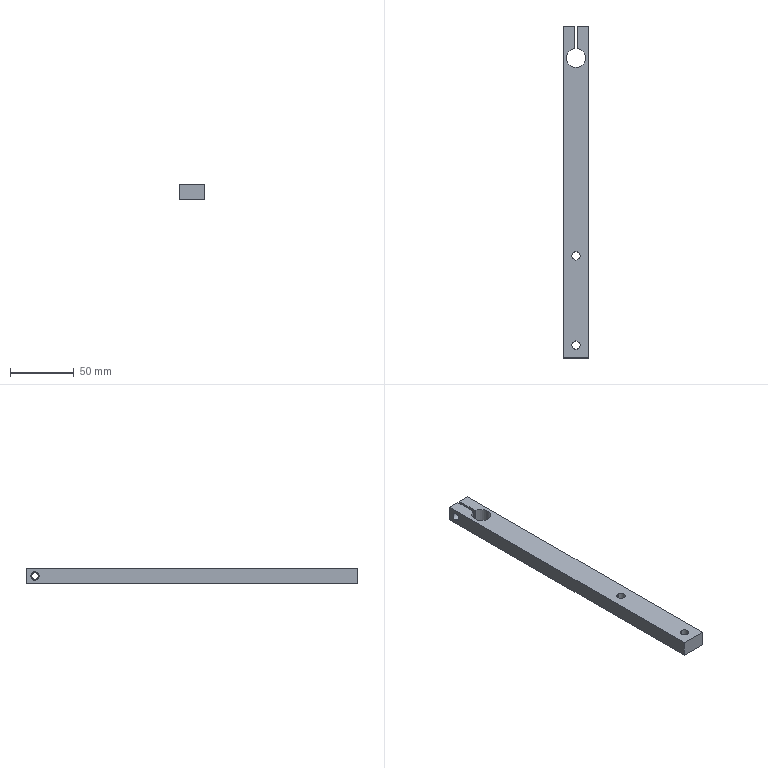Component | SolidWorks | KSD171005A-01-01-23-1 | 1 solid | 24 faces | box 20 x 260 x 12 mm | volume 57833 mm3 | cylinder 13 | plane 11 | commonest cylinder face diameters 11 x4 6.6 x4 6.5 x2 5 x2 15 x1
build123d program:
from build123d import *

# Parameters (mm, degrees)
SKETCH1_W                                       = 260
SKETCH1_H                                       = 20
BOSS_EXTRUDE1_DEPTH                             = 12
SKETCH2_R                                       = 7.5
CUT_EXTRUDE1_DEPTH                              = 131.935
SKETCH3_W                                       = 20
SKETCH3_H                                       = 2
CUT_EXTRUDE2_DEPTH                              = 131.935
M6_TAPPED_HOLE1_D                               = 5
F_6_5_6_5_DIAMETER_HOLE1_D                      = 6.5
F_6_5_6_5_DIAMETER_HOLE1_DEPTH                  = 10
F_6_5_6_5_DIAMETER_HOLE1_TIP                    = 1.953
M6_HEX_SOCKET_HEAD_CAP_SCREW_CBORE2_D           = 6.6
M6_HEX_SOCKET_HEAD_CAP_SCREW_CBORE2_CBORE_D     = 11
M6_HEX_SOCKET_HEAD_CAP_SCREW_CBORE2_CBORE_DEPTH = 6


with BuildPart() as part:
    # Sketch1 → Boss-Extrude1 (new body)
    with BuildSketch(Plane.XY):
        Rectangle(SKETCH1_W, SKETCH1_H)
    extrude(amount=BOSS_EXTRUDE1_DEPTH)

    # Sketch2 → Cut-Extrude1 (cut, through all)
    with BuildSketch(Plane.XY.offset(12)):
        with Locations((105, 0)):
            Circle(SKETCH2_R)
    extrude(amount=-CUT_EXTRUDE1_DEPTH, mode=Mode.SUBTRACT)

    # Sketch3 → Cut-Extrude2 (cut, through all)
    with BuildSketch(Plane.XY.offset(12)):
        with Locations((120, 0)):
            Rectangle(SKETCH3_W, SKETCH3_H)
    extrude(amount=-CUT_EXTRUDE2_DEPTH, mode=Mode.SUBTRACT)

    # M6 Tapped Hole1 (through all)
    with Locations(Plane(origin=(0, 10, 0), x_dir=(1, 0, 0), z_dir=(0, 1, 0))):
        with Locations((123, -6)):
            Hole(M6_TAPPED_HOLE1_D / 2)

    # 6.5 _6.5_ Diameter Hole1
    with Locations(Plane(origin=(0, 10, 0), x_dir=(1, 0, 0), z_dir=(0, 1, 0))):
        with Locations((123, -6)):
            Hole(F_6_5_6_5_DIAMETER_HOLE1_D / 2, depth=F_6_5_6_5_DIAMETER_HOLE1_DEPTH)
            with Locations((0, 0, -(F_6_5_6_5_DIAMETER_HOLE1_DEPTH + F_6_5_6_5_DIAMETER_HOLE1_TIP / 2))):  # 118° drill point
                Cone(0, F_6_5_6_5_DIAMETER_HOLE1_D / 2, F_6_5_6_5_DIAMETER_HOLE1_TIP, mode=Mode.SUBTRACT)

    # M6 Hex Socket Head Cap Screw CBORE2 (through all)
    with Locations(Plane(origin=(0, 0, 0), x_dir=(-1, 0, 0), z_dir=(0, 0, -1))):
        with Locations((120, 0), (50, 0)):
            CounterBoreHole(M6_HEX_SOCKET_HEAD_CAP_SCREW_CBORE2_D / 2, M6_HEX_SOCKET_HEAD_CAP_SCREW_CBORE2_CBORE_D / 2, M6_HEX_SOCKET_HEAD_CAP_SCREW_CBORE2_CBORE_DEPTH)


solid = part.part

# Placed as in the assembly
solid = solid.moved(Location((-7.111, -89.27, 616), (0, 0, 90)))
STEP:
#1=CARTESIAN_POINT('',(-0.28,-8.022,24.488));
#2=VERTEX_POINT('',#1);
#3=CARTESIAN_POINT('',(-0.28,-8.456,24.488));
#4=VERTEX_POINT('',#3);
#5=CARTESIAN_POINT('',(-0.28,-8.239,24.488));
#6=DIRECTION('',(0.,0.,-1.));
#7=DIRECTION('',(-0.,-1.,0.));
#8=AXIS2_PLACEMENT_3D('',#5,#6,#7);
#9=CIRCLE('',#8,0.2165);
#10=EDGE_CURVE('',#2,#4,#9,.T.);
#11=ORIENTED_EDGE('',*,*,#10,.F.);
#12=CARTESIAN_POINT('',(-0.28,-8.022,24.252));
#13=VERTEX_POINT('',#12);
#14=CARTESIAN_POINT('',(-0.28,-8.022,24.252));
#15=DIRECTION('',(0.,0.,-1.));
#16=VECTOR('',#15,39.37);
#17=LINE('',#14,#16);
#18=EDGE_CURVE('',#2,#13,#17,.T.);
#19=ORIENTED_EDGE('',*,*,#18,.T.);
#20=CARTESIAN_POINT('',(-0.28,-8.456,24.252));
#21=VERTEX_POINT('',#20);
#22=CARTESIAN_POINT('',(-0.28,-8.239,24.252));
#23=DIRECTION('',(0.,0.,-1.));
#24=DIRECTION('',(-0.,-1.,0.));
#25=AXIS2_PLACEMENT_3D('',#22,#23,#24);
#26=CIRCLE('',#25,0.2165);
#27=EDGE_CURVE('',#13,#21,#26,.T.);
#28=ORIENTED_EDGE('',*,*,#27,.T.);
#29=CARTESIAN_POINT('',(-0.28,-8.456,24.252));
#30=DIRECTION('',(0.,0.,-1.));
#31=VECTOR('',#30,39.37);
#32=LINE('',#29,#31);
#33=EDGE_CURVE('',#4,#21,#32,.T.);
#34=ORIENTED_EDGE('',*,*,#33,.F.);
#35=EDGE_LOOP('',(#11,#19,#28,#34));
#36=FACE_OUTER_BOUND('',#35,.T.);
#37=CARTESIAN_POINT('',(-0.28,-8.239,24.252));
#38=DIRECTION('',(0.,0.,-1.));
#39=DIRECTION('',(-0.,-1.,0.));
#40=AXIS2_PLACEMENT_3D('',#37,#38,#39);
#41=CYLINDRICAL_SURFACE('',#40,0.2165);
#42=ADVANCED_FACE('',(#36),#41,.F.);
#43=CARTESIAN_POINT('',(-0.28,-8.109,24.724));
#44=VERTEX_POINT('',#43);
#45=CARTESIAN_POINT('',(-0.28,-8.369,24.724));
#46=VERTEX_POINT('',#45);
#47=CARTESIAN_POINT('',(-0.28,-8.239,24.724));
#48=DIRECTION('',(0.,0.,-1.));
#49=DIRECTION('',(-0.,-1.,0.));
#50=AXIS2_PLACEMENT_3D('',#47,#48,#49);
#51=CIRCLE('',#50,0.1299);
#52=EDGE_CURVE('',#44,#46,#51,.T.);
#53=ORIENTED_EDGE('',*,*,#52,.F.);
#54=CARTESIAN_POINT('',(-0.28,-8.109,24.488));
#55=VERTEX_POINT('',#54);
#56=CARTESIAN_POINT('',(-0.28,-8.109,24.252));
#57=DIRECTION('',(0.,0.,-1.));
#58=VECTOR('',#57,39.37);
#59=LINE('',#56,#58);
#60=EDGE_CURVE('',#44,#55,#59,.T.);
#61=ORIENTED_EDGE('',*,*,#60,.T.);
#62=CARTESIAN_POINT('',(-0.28,-8.369,24.488));
#63=VERTEX_POINT('',#62);
#64=CARTESIAN_POINT('',(-0.28,-8.239,24.488));
#65=DIRECTION('',(0.,0.,-1.));
#66=DIRECTION('',(-0.,-1.,0.));
#67=AXIS2_PLACEMENT_3D('',#64,#65,#66);
#68=CIRCLE('',#67,0.1299);
#69=EDGE_CURVE('',#55,#63,#68,.T.);
#70=ORIENTED_EDGE('',*,*,#69,.T.);
#71=CARTESIAN_POINT('',(-0.28,-8.369,24.252));
#72=DIRECTION('',(0.,0.,-1.));
#73=VECTOR('',#72,39.37);
#74=LINE('',#71,#73);
#75=EDGE_CURVE('',#46,#63,#74,.T.);
#76=ORIENTED_EDGE('',*,*,#75,.F.);
#77=EDGE_LOOP('',(#53,#61,#70,#76));
#78=FACE_OUTER_BOUND('',#77,.T.);
#79=CARTESIAN_POINT('',(-0.28,-8.239,24.252));
#80=DIRECTION('',(0.,0.,-1.));
#81=DIRECTION('',(-0.,-1.,0.));
#82=AXIS2_PLACEMENT_3D('',#79,#80,#81);
#83=CYLINDRICAL_SURFACE('',#82,0.1299);
#84=ADVANCED_FACE('',(#78),#83,.F.);
#85=CARTESIAN_POINT('',(-0.28,-5.267,24.488));
#86=VERTEX_POINT('',#85);
#87=CARTESIAN_POINT('',(-0.28,-5.7,24.488));
#88=VERTEX_POINT('',#87);
#89=CARTESIAN_POINT('',(-0.28,-5.483,24.488));
#90=DIRECTION('',(0.,0.,-1.));
#91=DIRECTION('',(-0.,-1.,0.));
#92=AXIS2_PLACEMENT_3D('',#89,#90,#91);
#93=CIRCLE('',#92,0.2165);
#94=EDGE_CURVE('',#86,#88,#93,.T.);
#95=ORIENTED_EDGE('',*,*,#94,.F.);
#96=CARTESIAN_POINT('',(-0.28,-5.267,24.252));
#97=VERTEX_POINT('',#96);
#98=CARTESIAN_POINT('',(-0.28,-5.267,24.252));
#99=DIRECTION('',(0.,0.,-1.));
#100=VECTOR('',#99,39.37);
#101=LINE('',#98,#100);
#102=EDGE_CURVE('',#86,#97,#101,.T.);
#103=ORIENTED_EDGE('',*,*,#102,.T.);
#104=CARTESIAN_POINT('',(-0.28,-5.7,24.252));
#105=VERTEX_POINT('',#104);
#106=CARTESIAN_POINT('',(-0.28,-5.483,24.252));
#107=DIRECTION('',(0.,0.,-1.));
#108=DIRECTION('',(-0.,-1.,0.));
#109=AXIS2_PLACEMENT_3D('',#106,#107,#108);
#110=CIRCLE('',#109,0.2165);
#111=EDGE_CURVE('',#97,#105,#110,.T.);
#112=ORIENTED_EDGE('',*,*,#111,.T.);
#113=CARTESIAN_POINT('',(-0.28,-5.7,24.252));
#114=DIRECTION('',(0.,0.,-1.));
#115=VECTOR('',#114,39.37);
#116=LINE('',#113,#115);
#117=EDGE_CURVE('',#88,#105,#116,.T.);
#118=ORIENTED_EDGE('',*,*,#117,.F.);
#119=EDGE_LOOP('',(#95,#103,#112,#118));
#120=FACE_OUTER_BOUND('',#119,.T.);
#121=CARTESIAN_POINT('',(-0.28,-5.483,24.252));
#122=DIRECTION('',(0.,0.,-1.));
#123=DIRECTION('',(-0.,-1.,0.));
#124=AXIS2_PLACEMENT_3D('',#121,#122,#123);
#125=CYLINDRICAL_SURFACE('',#124,0.2165);
#126=ADVANCED_FACE('',(#120),#125,.F.);
#127=CARTESIAN_POINT('',(-0.28,-5.353,24.724));
#128=VERTEX_POINT('',#127);
#129=CARTESIAN_POINT('',(-0.28,-5.613,24.724));
#130=VERTEX_POINT('',#129);
#131=CARTESIAN_POINT('',(-0.28,-5.483,24.724));
#132=DIRECTION('',(0.,0.,-1.));
#133=DIRECTION('',(-0.,-1.,0.));
#134=AXIS2_PLACEMENT_3D('',#131,#132,#133);
#135=CIRCLE('',#134,0.1299);
#136=EDGE_CURVE('',#128,#130,#135,.T.);
#137=ORIENTED_EDGE('',*,*,#136,.F.);
#138=CARTESIAN_POINT('',(-0.28,-5.353,24.488));
#139=VERTEX_POINT('',#138);
#140=CARTESIAN_POINT('',(-0.28,-5.353,24.252));
#141=DIRECTION('',(0.,0.,-1.));
#142=VECTOR('',#141,39.37);
#143=LINE('',#140,#142);
#144=EDGE_CURVE('',#128,#139,#143,.T.);
#145=ORIENTED_EDGE('',*,*,#144,.T.);
#146=CARTESIAN_POINT('',(-0.28,-5.613,24.488));
#147=VERTEX_POINT('',#146);
#148=CARTESIAN_POINT('',(-0.28,-5.483,24.488));
#149=DIRECTION('',(0.,0.,-1.));
#150=DIRECTION('',(-0.,-1.,0.));
#151=AXIS2_PLACEMENT_3D('',#148,#149,#150);
#152=CIRCLE('',#151,0.1299);
#153=EDGE_CURVE('',#139,#147,#152,.T.);
#154=ORIENTED_EDGE('',*,*,#153,.T.);
#155=CARTESIAN_POINT('',(-0.28,-5.613,24.252));
#156=DIRECTION('',(0.,0.,-1.));
#157=VECTOR('',#156,39.37);
#158=LINE('',#155,#157);
#159=EDGE_CURVE('',#130,#147,#158,.T.);
#160=ORIENTED_EDGE('',*,*,#159,.F.);
#161=EDGE_LOOP('',(#137,#145,#154,#160));
#162=FACE_OUTER_BOUND('',#161,.T.);
#163=CARTESIAN_POINT('',(-0.28,-5.483,24.252));
#164=DIRECTION('',(0.,0.,-1.));
#165=DIRECTION('',(-0.,-1.,0.));
#166=AXIS2_PLACEMENT_3D('',#163,#164,#165);
#167=CYLINDRICAL_SURFACE('',#166,0.1299);
#168=ADVANCED_FACE('',(#162),#167,.F.);
#169=CARTESIAN_POINT('',(-0.3193,1.328,24.36));
#170=VERTEX_POINT('',#169);
#171=CARTESIAN_POINT('',(-0.3193,1.328,24.616));
#172=VERTEX_POINT('',#171);
#173=CARTESIAN_POINT('',(-0.3193,1.328,24.488));
#174=DIRECTION('',(-1.,0.,0.));
#175=DIRECTION('',(0.,-1.,0.));
#176=AXIS2_PLACEMENT_3D('',#173,#174,#175);
#177=CIRCLE('',#176,0.128);
#178=EDGE_CURVE('',#170,#172,#177,.T.);
#179=ORIENTED_EDGE('',*,*,#178,.F.);
#180=CARTESIAN_POINT('',(-0.6737,1.328,24.36));
#181=VERTEX_POINT('',#180);
#182=CARTESIAN_POINT('',(-0.6737,1.328,24.36));
#183=DIRECTION('',(-1.,0.,0.));
#184=VECTOR('',#183,39.37);
#185=LINE('',#182,#184);
#186=EDGE_CURVE('',#170,#181,#185,.T.);
#187=ORIENTED_EDGE('',*,*,#186,.T.);
#188=CARTESIAN_POINT('',(-0.6737,1.328,24.616));
#189=VERTEX_POINT('',#188);
#190=CARTESIAN_POINT('',(-0.6737,1.328,24.488));
#191=DIRECTION('',(-1.,0.,0.));
#192=DIRECTION('',(0.,0.,1.));
#193=AXIS2_PLACEMENT_3D('',#190,#191,#192);
#194=CIRCLE('',#193,0.128);
#195=EDGE_CURVE('',#181,#189,#194,.T.);
#196=ORIENTED_EDGE('',*,*,#195,.T.);
#197=CARTESIAN_POINT('',(-0.6737,1.328,24.616));
#198=DIRECTION('',(-1.,0.,0.));
#199=VECTOR('',#198,39.37);
#200=LINE('',#197,#199);
#201=EDGE_CURVE('',#172,#189,#200,.T.);
#202=ORIENTED_EDGE('',*,*,#201,.F.);
#203=EDGE_LOOP('',(#179,#187,#196,#202));
#204=FACE_OUTER_BOUND('',#203,.T.);
#205=CARTESIAN_POINT('',(-0.6737,1.328,24.488));
#206=DIRECTION('',(-1.,0.,0.));
#207=DIRECTION('',(0.,0.,1.));
#208=AXIS2_PLACEMENT_3D('',#205,#206,#207);
#209=CYLINDRICAL_SURFACE('',#208,0.128);
#210=ADVANCED_FACE('',(#204),#209,.F.);
#211=CARTESIAN_POINT('',(0.1137,1.328,24.39));
#212=VERTEX_POINT('',#211);
#213=CARTESIAN_POINT('',(0.1137,1.328,24.587));
#214=VERTEX_POINT('',#213);
#215=CARTESIAN_POINT('',(0.1137,1.328,24.488));
#216=DIRECTION('',(-1.,0.,0.));
#217=DIRECTION('',(0.,0.,1.));
#218=AXIS2_PLACEMENT_3D('',#215,#216,#217);
#219=CIRCLE('',#218,0.09843);
#220=EDGE_CURVE('',#212,#214,#219,.T.);
#221=ORIENTED_EDGE('',*,*,#220,.F.);
#222=CARTESIAN_POINT('',(-0.2406,1.328,24.39));
#223=VERTEX_POINT('',#222);
#224=CARTESIAN_POINT('',(-0.6737,1.328,24.39));
#225=DIRECTION('',(-1.,0.,0.));
#226=VECTOR('',#225,39.37);
#227=LINE('',#224,#226);
#228=EDGE_CURVE('',#212,#223,#227,.T.);
#229=ORIENTED_EDGE('',*,*,#228,.T.);
#230=CARTESIAN_POINT('',(-0.2406,1.328,24.587));
#231=VERTEX_POINT('',#230);
#232=CARTESIAN_POINT('',(-0.2406,1.328,24.488));
#233=DIRECTION('',(1.,-0.,0.));
#234=DIRECTION('',(0.,1.,0.));
#235=AXIS2_PLACEMENT_3D('',#232,#233,#234);
#236=CIRCLE('',#235,0.09843);
#237=EDGE_CURVE('',#231,#223,#236,.T.);
#238=ORIENTED_EDGE('',*,*,#237,.F.);
#239=CARTESIAN_POINT('',(-0.6737,1.328,24.587));
#240=DIRECTION('',(-1.,0.,0.));
#241=VECTOR('',#240,39.37);
#242=LINE('',#239,#241);
#243=EDGE_CURVE('',#214,#231,#242,.T.);
#244=ORIENTED_EDGE('',*,*,#243,.F.);
#245=EDGE_LOOP('',(#221,#229,#238,#244));
#246=FACE_OUTER_BOUND('',#245,.T.);
#247=CARTESIAN_POINT('',(-0.6737,1.328,24.488));
#248=DIRECTION('',(-1.,0.,0.));
#249=DIRECTION('',(0.,0.,1.));
#250=AXIS2_PLACEMENT_3D('',#247,#248,#249);
#251=CYLINDRICAL_SURFACE('',#250,0.09843);
#252=ADVANCED_FACE('',(#246),#251,.F.);
#253=CARTESIAN_POINT('',(-0.3193,1.604,24.724));
#254=VERTEX_POINT('',#253);
#255=CARTESIAN_POINT('',(-0.6737,1.604,24.724));
#256=VERTEX_POINT('',#255);
#257=CARTESIAN_POINT('',(-0.6737,1.604,24.724));
#258=DIRECTION('',(-1.,0.,0.));
#259=VECTOR('',#258,39.37);
#260=LINE('',#257,#259);
#261=EDGE_CURVE('',#254,#256,#260,.T.);
#262=ORIENTED_EDGE('',*,*,#261,.F.);
#263=CARTESIAN_POINT('',(-0.3193,1.604,24.252));
#264=VERTEX_POINT('',#263);
#265=CARTESIAN_POINT('',(-0.3193,1.604,24.252));
#266=DIRECTION('',(0.,0.,1.));
#267=VECTOR('',#266,39.37);
#268=LINE('',#265,#267);
#269=EDGE_CURVE('',#264,#254,#268,.T.);
#270=ORIENTED_EDGE('',*,*,#269,.F.);
#271=CARTESIAN_POINT('',(-0.6737,1.604,24.252));
#272=VERTEX_POINT('',#271);
#273=CARTESIAN_POINT('',(-0.6737,1.604,24.252));
#274=DIRECTION('',(-1.,0.,0.));
#275=VECTOR('',#274,39.37);
#276=LINE('',#273,#275);
#277=EDGE_CURVE('',#264,#272,#276,.T.);
#278=ORIENTED_EDGE('',*,*,#277,.T.);
#279=CARTESIAN_POINT('',(-0.6737,1.604,24.724));
#280=DIRECTION('',(0.,0.,-1.));
#281=VECTOR('',#280,39.37);
#282=LINE('',#279,#281);
#283=EDGE_CURVE('',#256,#272,#282,.T.);
#284=ORIENTED_EDGE('',*,*,#283,.F.);
#285=EDGE_LOOP('',(#262,#270,#278,#284));
#286=FACE_OUTER_BOUND('',#285,.T.);
#287=CARTESIAN_POINT('',(-0.6737,1.604,24.724));
#288=DIRECTION('',(-0.,-1.,0.));
#289=DIRECTION('',(0.,0.,1.));
#290=AXIS2_PLACEMENT_3D('',#287,#288,#289);
#291=PLANE('',#290);
#292=ADVANCED_FACE('',(#286),#291,.F.);
#293=CARTESIAN_POINT('',(0.1137,1.604,24.252));
#294=VERTEX_POINT('',#293);
#295=CARTESIAN_POINT('',(-0.2406,1.604,24.252));
#296=VERTEX_POINT('',#295);
#297=CARTESIAN_POINT('',(-0.6737,1.604,24.252));
#298=DIRECTION('',(-1.,0.,0.));
#299=VECTOR('',#298,39.37);
#300=LINE('',#297,#299);
#301=EDGE_CURVE('',#294,#296,#300,.T.);
#302=ORIENTED_EDGE('',*,*,#301,.T.);
#303=CARTESIAN_POINT('',(-0.2406,1.604,24.724));
#304=VERTEX_POINT('',#303);
#305=CARTESIAN_POINT('',(-0.2406,1.604,24.252));
#306=DIRECTION('',(0.,0.,1.));
#307=VECTOR('',#306,39.37);
#308=LINE('',#305,#307);
#309=EDGE_CURVE('',#296,#304,#308,.T.);
#310=ORIENTED_EDGE('',*,*,#309,.T.);
#311=CARTESIAN_POINT('',(0.1137,1.604,24.724));
#312=VERTEX_POINT('',#311);
#313=CARTESIAN_POINT('',(-0.6737,1.604,24.724));
#314=DIRECTION('',(-1.,0.,0.));
#315=VECTOR('',#314,39.37);
#316=LINE('',#313,#315);
#317=EDGE_CURVE('',#312,#304,#316,.T.);
#318=ORIENTED_EDGE('',*,*,#317,.F.);
#319=CARTESIAN_POINT('',(0.1137,1.604,24.724));
#320=DIRECTION('',(0.,0.,-1.));
#321=VECTOR('',#320,39.37);
#322=LINE('',#319,#321);
#323=EDGE_CURVE('',#312,#294,#322,.T.);
#324=ORIENTED_EDGE('',*,*,#323,.T.);
#325=EDGE_LOOP('',(#302,#310,#318,#324));
#326=FACE_OUTER_BOUND('',#325,.T.);
#327=CARTESIAN_POINT('',(-0.6737,1.604,24.724));
#328=DIRECTION('',(-0.,-1.,0.));
#329=DIRECTION('',(0.,0.,1.));
#330=AXIS2_PLACEMENT_3D('',#327,#328,#329);
#331=PLANE('',#330);
#332=ADVANCED_FACE('',(#326),#331,.F.);
#333=CARTESIAN_POINT('',(-0.6737,1.328,24.488));
#334=DIRECTION('',(-1.,0.,0.));
#335=DIRECTION('',(0.,0.,1.));
#336=AXIS2_PLACEMENT_3D('',#333,#334,#335);
#337=CIRCLE('',#336,0.128);
#338=EDGE_CURVE('',#189,#181,#337,.T.);
#339=ORIENTED_EDGE('',*,*,#338,.F.);
#340=ORIENTED_EDGE('',*,*,#195,.F.);
#341=EDGE_LOOP('',(#339,#340));
#342=FACE_BOUND('',#341,.T.);
#343=CARTESIAN_POINT('',(-0.6737,-8.633,24.252));
#344=VERTEX_POINT('',#343);
#345=CARTESIAN_POINT('',(-0.6737,-8.633,24.252));
#346=DIRECTION('',(-0.,-1.,0.));
#347=VECTOR('',#346,39.37);
#348=LINE('',#345,#347);
#349=EDGE_CURVE('',#272,#344,#348,.T.);
#350=ORIENTED_EDGE('',*,*,#349,.T.);
#351=CARTESIAN_POINT('',(-0.6737,-8.633,24.724));
#352=VERTEX_POINT('',#351);
#353=CARTESIAN_POINT('',(-0.6737,-8.633,24.724));
#354=DIRECTION('',(0.,0.,-1.));
#355=VECTOR('',#354,39.37);
#356=LINE('',#353,#355);
#357=EDGE_CURVE('',#352,#344,#356,.T.);
#358=ORIENTED_EDGE('',*,*,#357,.F.);
#359=CARTESIAN_POINT('',(-0.6737,-8.633,24.724));
#360=DIRECTION('',(-0.,-1.,0.));
#361=VECTOR('',#360,39.37);
#362=LINE('',#359,#361);
#363=EDGE_CURVE('',#256,#352,#362,.T.);
#364=ORIENTED_EDGE('',*,*,#363,.F.);
#365=ORIENTED_EDGE('',*,*,#283,.T.);
#366=EDGE_LOOP('',(#350,#358,#364,#365));
#367=FACE_OUTER_BOUND('',#366,.T.);
#368=CARTESIAN_POINT('',(-0.6737,-8.633,24.724));
#369=DIRECTION('',(1.,-0.,0.));
#370=DIRECTION('',(0.,0.,-1.));
#371=AXIS2_PLACEMENT_3D('',#368,#369,#370);
#372=PLANE('',#371);
#373=ADVANCED_FACE('',(#342,#367),#372,.F.);
#374=CARTESIAN_POINT('',(0.1137,-8.633,24.252));
#375=VERTEX_POINT('',#374);
#376=CARTESIAN_POINT('',(-0.6737,-8.633,24.252));
#377=DIRECTION('',(1.,-0.,0.));
#378=VECTOR('',#377,39.37);
#379=LINE('',#376,#378);
#380=EDGE_CURVE('',#344,#375,#379,.T.);
#381=ORIENTED_EDGE('',*,*,#380,.T.);
#382=CARTESIAN_POINT('',(0.1137,-8.633,24.724));
#383=VERTEX_POINT('',#382);
#384=CARTESIAN_POINT('',(0.1137,-8.633,24.724));
#385=DIRECTION('',(0.,0.,-1.));
#386=VECTOR('',#385,39.37);
#387=LINE('',#384,#386);
#388=EDGE_CURVE('',#383,#375,#387,.T.);
#389=ORIENTED_EDGE('',*,*,#388,.F.);
#390=CARTESIAN_POINT('',(-0.6737,-8.633,24.724));
#391=DIRECTION('',(1.,-0.,0.));
#392=VECTOR('',#391,39.37);
#393=LINE('',#390,#392);
#394=EDGE_CURVE('',#352,#383,#393,.T.);
#395=ORIENTED_EDGE('',*,*,#394,.F.);
#396=ORIENTED_EDGE('',*,*,#357,.T.);
#397=EDGE_LOOP('',(#381,#389,#395,#396));
#398=FACE_OUTER_BOUND('',#397,.T.);
#399=CARTESIAN_POINT('',(-0.6737,-8.633,24.724));
#400=DIRECTION('',(0.,1.,0.));
#401=DIRECTION('',(0.,0.,-1.));
#402=AXIS2_PLACEMENT_3D('',#399,#400,#401);
#403=PLANE('',#402);
#404=ADVANCED_FACE('',(#398),#403,.F.);
#405=CARTESIAN_POINT('',(0.1137,1.328,24.488));
#406=DIRECTION('',(-1.,0.,0.));
#407=DIRECTION('',(0.,0.,1.));
#408=AXIS2_PLACEMENT_3D('',#405,#406,#407);
#409=CIRCLE('',#408,0.09843);
#410=EDGE_CURVE('',#214,#212,#409,.T.);
#411=ORIENTED_EDGE('',*,*,#410,.T.);
#412=ORIENTED_EDGE('',*,*,#220,.T.);
#413=EDGE_LOOP('',(#411,#412));
#414=FACE_BOUND('',#413,.T.);
#415=CARTESIAN_POINT('',(0.1137,-8.633,24.252));
#416=DIRECTION('',(0.,1.,0.));
#417=VECTOR('',#416,39.37);
#418=LINE('',#415,#417);
#419=EDGE_CURVE('',#375,#294,#418,.T.);
#420=ORIENTED_EDGE('',*,*,#419,.T.);
#421=ORIENTED_EDGE('',*,*,#323,.F.);
#422=CARTESIAN_POINT('',(0.1137,-8.633,24.724));
#423=DIRECTION('',(0.,1.,0.));
#424=VECTOR('',#423,39.37);
#425=LINE('',#422,#424);
#426=EDGE_CURVE('',#383,#312,#425,.T.);
#427=ORIENTED_EDGE('',*,*,#426,.F.);
#428=ORIENTED_EDGE('',*,*,#388,.T.);
#429=EDGE_LOOP('',(#420,#421,#427,#428));
#430=FACE_OUTER_BOUND('',#429,.T.);
#431=CARTESIAN_POINT('',(0.1137,-8.633,24.724));
#432=DIRECTION('',(-1.,0.,0.));
#433=DIRECTION('',(0.,0.,1.));
#434=AXIS2_PLACEMENT_3D('',#431,#432,#433);
#435=PLANE('',#434);
#436=ADVANCED_FACE('',(#414,#430),#435,.F.);
#437=CARTESIAN_POINT('',(-0.28,-8.239,24.724));
#438=DIRECTION('',(0.,0.,-1.));
#439=DIRECTION('',(-0.,-1.,0.));
#440=AXIS2_PLACEMENT_3D('',#437,#438,#439);
#441=CIRCLE('',#440,0.1299);
#442=EDGE_CURVE('',#46,#44,#441,.T.);
#443=ORIENTED_EDGE('',*,*,#442,.T.);
#444=ORIENTED_EDGE('',*,*,#52,.T.);
#445=EDGE_LOOP('',(#443,#444));
#446=FACE_BOUND('',#445,.T.);
#447=CARTESIAN_POINT('',(-0.28,-5.483,24.724));
#448=DIRECTION('',(0.,0.,-1.));
#449=DIRECTION('',(-0.,-1.,0.));
#450=AXIS2_PLACEMENT_3D('',#447,#448,#449);
#451=CIRCLE('',#450,0.1299);
#452=EDGE_CURVE('',#130,#128,#451,.T.);
#453=ORIENTED_EDGE('',*,*,#452,.T.);
#454=ORIENTED_EDGE('',*,*,#136,.T.);
#455=EDGE_LOOP('',(#453,#454));
#456=FACE_BOUND('',#455,.T.);
#457=CARTESIAN_POINT('',(-0.3193,0.9119,24.724));
#458=VERTEX_POINT('',#457);
#459=CARTESIAN_POINT('',(-0.3193,0.8161,24.724));
#460=DIRECTION('',(-0.,-1.,0.));
#461=VECTOR('',#460,39.37);
#462=LINE('',#459,#461);
#463=EDGE_CURVE('',#254,#458,#462,.T.);
#464=ORIENTED_EDGE('',*,*,#463,.F.);
#465=ORIENTED_EDGE('',*,*,#261,.T.);
#466=ORIENTED_EDGE('',*,*,#363,.T.);
#467=ORIENTED_EDGE('',*,*,#394,.T.);
#468=ORIENTED_EDGE('',*,*,#426,.T.);
#469=ORIENTED_EDGE('',*,*,#317,.T.);
#470=CARTESIAN_POINT('',(-0.2406,0.9119,24.724));
#471=VERTEX_POINT('',#470);
#472=CARTESIAN_POINT('',(-0.2406,0.8161,24.724));
#473=DIRECTION('',(0.,1.,0.));
#474=VECTOR('',#473,39.37);
#475=LINE('',#472,#474);
#476=EDGE_CURVE('',#471,#304,#475,.T.);
#477=ORIENTED_EDGE('',*,*,#476,.F.);
#478=CARTESIAN_POINT('',(-0.28,0.6193,24.724));
#479=DIRECTION('',(0.,0.,1.));
#480=DIRECTION('',(0.,1.,0.));
#481=AXIS2_PLACEMENT_3D('',#478,#479,#480);
#482=CIRCLE('',#481,0.2953);
#483=EDGE_CURVE('',#458,#471,#482,.T.);
#484=ORIENTED_EDGE('',*,*,#483,.F.);
#485=EDGE_LOOP('',(#464,#465,#466,#467,#468,#469,#477,#484));
#486=FACE_OUTER_BOUND('',#485,.T.);
#487=CARTESIAN_POINT('',(-0.28,-3.515,24.724));
#488=DIRECTION('',(0.,0.,1.));
#489=DIRECTION('',(0.,1.,0.));
#490=AXIS2_PLACEMENT_3D('',#487,#488,#489);
#491=PLANE('',#490);
#492=ADVANCED_FACE('',(#446,#456,#486),#491,.T.);
#493=CARTESIAN_POINT('',(-0.28,-8.239,24.252));
#494=DIRECTION('',(0.,0.,-1.));
#495=DIRECTION('',(-0.,-1.,0.));
#496=AXIS2_PLACEMENT_3D('',#493,#494,#495);
#497=CIRCLE('',#496,0.2165);
#498=EDGE_CURVE('',#21,#13,#497,.T.);
#499=ORIENTED_EDGE('',*,*,#498,.F.);
#500=ORIENTED_EDGE('',*,*,#27,.F.);
#501=EDGE_LOOP('',(#499,#500));
#502=FACE_BOUND('',#501,.T.);
#503=CARTESIAN_POINT('',(-0.28,-5.483,24.252));
#504=DIRECTION('',(0.,0.,-1.));
#505=DIRECTION('',(-0.,-1.,0.));
#506=AXIS2_PLACEMENT_3D('',#503,#504,#505);
#507=CIRCLE('',#506,0.2165);
#508=EDGE_CURVE('',#105,#97,#507,.T.);
#509=ORIENTED_EDGE('',*,*,#508,.F.);
#510=ORIENTED_EDGE('',*,*,#111,.F.);
#511=EDGE_LOOP('',(#509,#510));
#512=FACE_BOUND('',#511,.T.);
#513=ORIENTED_EDGE('',*,*,#277,.F.);
#514=CARTESIAN_POINT('',(-0.3193,0.9119,24.252));
#515=VERTEX_POINT('',#514);
#516=CARTESIAN_POINT('',(-0.3193,0.8161,24.252));
#517=DIRECTION('',(-0.,-1.,0.));
#518=VECTOR('',#517,39.37);
#519=LINE('',#516,#518);
#520=EDGE_CURVE('',#264,#515,#519,.T.);
#521=ORIENTED_EDGE('',*,*,#520,.T.);
#522=CARTESIAN_POINT('',(-0.2406,0.9119,24.252));
#523=VERTEX_POINT('',#522);
#524=CARTESIAN_POINT('',(-0.28,0.6193,24.252));
#525=DIRECTION('',(0.,0.,1.));
#526=DIRECTION('',(0.,1.,0.));
#527=AXIS2_PLACEMENT_3D('',#524,#525,#526);
#528=CIRCLE('',#527,0.2953);
#529=EDGE_CURVE('',#515,#523,#528,.T.);
#530=ORIENTED_EDGE('',*,*,#529,.T.);
#531=CARTESIAN_POINT('',(-0.2406,0.8161,24.252));
#532=DIRECTION('',(0.,1.,0.));
#533=VECTOR('',#532,39.37);
#534=LINE('',#531,#533);
#535=EDGE_CURVE('',#523,#296,#534,.T.);
#536=ORIENTED_EDGE('',*,*,#535,.T.);
#537=ORIENTED_EDGE('',*,*,#301,.F.);
#538=ORIENTED_EDGE('',*,*,#419,.F.);
#539=ORIENTED_EDGE('',*,*,#380,.F.);
#540=ORIENTED_EDGE('',*,*,#349,.F.);
#541=EDGE_LOOP('',(#513,#521,#530,#536,#537,#538,#539,#540));
#542=FACE_OUTER_BOUND('',#541,.T.);
#543=CARTESIAN_POINT('',(-0.28,-3.515,24.252));
#544=DIRECTION('',(0.,0.,1.));
#545=DIRECTION('',(0.,1.,0.));
#546=AXIS2_PLACEMENT_3D('',#543,#544,#545);
#547=PLANE('',#546);
#548=ADVANCED_FACE('',(#502,#512,#542),#547,.F.);
#549=ORIENTED_EDGE('',*,*,#529,.F.);
#550=CARTESIAN_POINT('',(-0.3193,0.9119,24.252));
#551=DIRECTION('',(0.,0.,1.));
#552=VECTOR('',#551,39.37);
#553=LINE('',#550,#552);
#554=EDGE_CURVE('',#515,#458,#553,.T.);
#555=ORIENTED_EDGE('',*,*,#554,.T.);
#556=ORIENTED_EDGE('',*,*,#483,.T.);
#557=CARTESIAN_POINT('',(-0.2406,0.9119,24.252));
#558=DIRECTION('',(0.,0.,-1.));
#559=VECTOR('',#558,39.37);
#560=LINE('',#557,#559);
#561=EDGE_CURVE('',#471,#523,#560,.T.);
#562=ORIENTED_EDGE('',*,*,#561,.T.);
#563=EDGE_LOOP('',(#549,#555,#556,#562));
#564=FACE_OUTER_BOUND('',#563,.T.);
#565=CARTESIAN_POINT('',(-0.28,0.6193,24.252));
#566=DIRECTION('',(0.,0.,1.));
#567=DIRECTION('',(0.,1.,0.));
#568=AXIS2_PLACEMENT_3D('',#565,#566,#567);
#569=CYLINDRICAL_SURFACE('',#568,0.2953);
#570=ADVANCED_FACE('',(#564),#569,.F.);
#571=ORIENTED_EDGE('',*,*,#237,.T.);
#572=CARTESIAN_POINT('',(-0.2406,1.328,24.488));
#573=DIRECTION('',(1.,-0.,0.));
#574=DIRECTION('',(0.,1.,0.));
#575=AXIS2_PLACEMENT_3D('',#572,#573,#574);
#576=CIRCLE('',#575,0.09843);
#577=EDGE_CURVE('',#223,#231,#576,.T.);
#578=ORIENTED_EDGE('',*,*,#577,.T.);
#579=EDGE_LOOP('',(#571,#578));
#580=FACE_BOUND('',#579,.T.);
#581=ORIENTED_EDGE('',*,*,#476,.T.);
#582=ORIENTED_EDGE('',*,*,#309,.F.);
#583=ORIENTED_EDGE('',*,*,#535,.F.);
#584=ORIENTED_EDGE('',*,*,#561,.F.);
#585=EDGE_LOOP('',(#581,#582,#583,#584));
#586=FACE_OUTER_BOUND('',#585,.T.);
#587=CARTESIAN_POINT('',(-0.2406,0.8161,24.252));
#588=DIRECTION('',(1.,-0.,0.));
#589=DIRECTION('',(0.,1.,0.));
#590=AXIS2_PLACEMENT_3D('',#587,#588,#589);
#591=PLANE('',#590);
#592=ADVANCED_FACE('',(#580,#586),#591,.F.);
#593=CARTESIAN_POINT('',(-0.3193,1.328,24.488));
#594=DIRECTION('',(-1.,0.,0.));
#595=DIRECTION('',(0.,-1.,0.));
#596=AXIS2_PLACEMENT_3D('',#593,#594,#595);
#597=CIRCLE('',#596,0.128);
#598=EDGE_CURVE('',#172,#170,#597,.T.);
#599=ORIENTED_EDGE('',*,*,#598,.T.);
#600=ORIENTED_EDGE('',*,*,#178,.T.);
#601=EDGE_LOOP('',(#599,#600));
#602=FACE_BOUND('',#601,.T.);
#603=ORIENTED_EDGE('',*,*,#520,.F.);
#604=ORIENTED_EDGE('',*,*,#269,.T.);
#605=ORIENTED_EDGE('',*,*,#463,.T.);
#606=ORIENTED_EDGE('',*,*,#554,.F.);
#607=EDGE_LOOP('',(#603,#604,#605,#606));
#608=FACE_OUTER_BOUND('',#607,.T.);
#609=CARTESIAN_POINT('',(-0.3193,0.8161,24.252));
#610=DIRECTION('',(-1.,0.,0.));
#611=DIRECTION('',(-0.,-1.,0.));
#612=AXIS2_PLACEMENT_3D('',#609,#610,#611);
#613=PLANE('',#612);
#614=ADVANCED_FACE('',(#602,#608),#613,.F.);
#615=ORIENTED_EDGE('',*,*,#228,.F.);
#616=ORIENTED_EDGE('',*,*,#410,.F.);
#617=ORIENTED_EDGE('',*,*,#243,.T.);
#618=ORIENTED_EDGE('',*,*,#577,.F.);
#619=EDGE_LOOP('',(#615,#616,#617,#618));
#620=FACE_OUTER_BOUND('',#619,.T.);
#621=CARTESIAN_POINT('',(-0.6737,1.328,24.488));
#622=DIRECTION('',(-1.,0.,0.));
#623=DIRECTION('',(0.,0.,1.));
#624=AXIS2_PLACEMENT_3D('',#621,#622,#623);
#625=CYLINDRICAL_SURFACE('',#624,0.09843);
#626=ADVANCED_FACE('',(#620),#625,.F.);
#627=ORIENTED_EDGE('',*,*,#186,.F.);
#628=ORIENTED_EDGE('',*,*,#598,.F.);
#629=ORIENTED_EDGE('',*,*,#201,.T.);
#630=ORIENTED_EDGE('',*,*,#338,.T.);
#631=EDGE_LOOP('',(#627,#628,#629,#630));
#632=FACE_OUTER_BOUND('',#631,.T.);
#633=CARTESIAN_POINT('',(-0.6737,1.328,24.488));
#634=DIRECTION('',(-1.,0.,0.));
#635=DIRECTION('',(0.,0.,1.));
#636=AXIS2_PLACEMENT_3D('',#633,#634,#635);
#637=CYLINDRICAL_SURFACE('',#636,0.128);
#638=ADVANCED_FACE('',(#632),#637,.F.);
#639=ORIENTED_EDGE('',*,*,#144,.F.);
#640=ORIENTED_EDGE('',*,*,#452,.F.);
#641=ORIENTED_EDGE('',*,*,#159,.T.);
#642=CARTESIAN_POINT('',(-0.28,-5.483,24.488));
#643=DIRECTION('',(0.,0.,-1.));
#644=DIRECTION('',(-0.,-1.,0.));
#645=AXIS2_PLACEMENT_3D('',#642,#643,#644);
#646=CIRCLE('',#645,0.1299);
#647=EDGE_CURVE('',#147,#139,#646,.T.);
#648=ORIENTED_EDGE('',*,*,#647,.T.);
#649=EDGE_LOOP('',(#639,#640,#641,#648));
#650=FACE_OUTER_BOUND('',#649,.T.);
#651=CARTESIAN_POINT('',(-0.28,-5.483,24.252));
#652=DIRECTION('',(0.,0.,-1.));
#653=DIRECTION('',(-0.,-1.,0.));
#654=AXIS2_PLACEMENT_3D('',#651,#652,#653);
#655=CYLINDRICAL_SURFACE('',#654,0.1299);
#656=ADVANCED_FACE('',(#650),#655,.F.);
#657=ORIENTED_EDGE('',*,*,#647,.F.);
#658=ORIENTED_EDGE('',*,*,#153,.F.);
#659=EDGE_LOOP('',(#657,#658));
#660=FACE_BOUND('',#659,.T.);
#661=CARTESIAN_POINT('',(-0.28,-5.483,24.488));
#662=DIRECTION('',(0.,0.,-1.));
#663=DIRECTION('',(-0.,-1.,0.));
#664=AXIS2_PLACEMENT_3D('',#661,#662,#663);
#665=CIRCLE('',#664,0.2165);
#666=EDGE_CURVE('',#88,#86,#665,.T.);
#667=ORIENTED_EDGE('',*,*,#666,.T.);
#668=ORIENTED_EDGE('',*,*,#94,.T.);
#669=EDGE_LOOP('',(#667,#668));
#670=FACE_OUTER_BOUND('',#669,.T.);
#671=CARTESIAN_POINT('',(-0.28,-5.353,24.488));
#672=DIRECTION('',(0.,0.,1.));
#673=DIRECTION('',(0.,1.,0.));
#674=AXIS2_PLACEMENT_3D('',#671,#672,#673);
#675=PLANE('',#674);
#676=ADVANCED_FACE('',(#660,#670),#675,.F.);
#677=ORIENTED_EDGE('',*,*,#102,.F.);
#678=ORIENTED_EDGE('',*,*,#666,.F.);
#679=ORIENTED_EDGE('',*,*,#117,.T.);
#680=ORIENTED_EDGE('',*,*,#508,.T.);
#681=EDGE_LOOP('',(#677,#678,#679,#680));
#682=FACE_OUTER_BOUND('',#681,.T.);
#683=CARTESIAN_POINT('',(-0.28,-5.483,24.252));
#684=DIRECTION('',(0.,0.,-1.));
#685=DIRECTION('',(-0.,-1.,0.));
#686=AXIS2_PLACEMENT_3D('',#683,#684,#685);
#687=CYLINDRICAL_SURFACE('',#686,0.2165);
#688=ADVANCED_FACE('',(#682),#687,.F.);
#689=ORIENTED_EDGE('',*,*,#60,.F.);
#690=ORIENTED_EDGE('',*,*,#442,.F.);
#691=ORIENTED_EDGE('',*,*,#75,.T.);
#692=CARTESIAN_POINT('',(-0.28,-8.239,24.488));
#693=DIRECTION('',(0.,0.,-1.));
#694=DIRECTION('',(-0.,-1.,0.));
#695=AXIS2_PLACEMENT_3D('',#692,#693,#694);
#696=CIRCLE('',#695,0.1299);
#697=EDGE_CURVE('',#63,#55,#696,.T.);
#698=ORIENTED_EDGE('',*,*,#697,.T.);
#699=EDGE_LOOP('',(#689,#690,#691,#698));
#700=FACE_OUTER_BOUND('',#699,.T.);
#701=CARTESIAN_POINT('',(-0.28,-8.239,24.252));
#702=DIRECTION('',(0.,0.,-1.));
#703=DIRECTION('',(-0.,-1.,0.));
#704=AXIS2_PLACEMENT_3D('',#701,#702,#703);
#705=CYLINDRICAL_SURFACE('',#704,0.1299);
#706=ADVANCED_FACE('',(#700),#705,.F.);
#707=ORIENTED_EDGE('',*,*,#697,.F.);
#708=ORIENTED_EDGE('',*,*,#69,.F.);
#709=EDGE_LOOP('',(#707,#708));
#710=FACE_BOUND('',#709,.T.);
#711=CARTESIAN_POINT('',(-0.28,-8.239,24.488));
#712=DIRECTION('',(0.,0.,-1.));
#713=DIRECTION('',(-0.,-1.,0.));
#714=AXIS2_PLACEMENT_3D('',#711,#712,#713);
#715=CIRCLE('',#714,0.2165);
#716=EDGE_CURVE('',#4,#2,#715,.T.);
#717=ORIENTED_EDGE('',*,*,#716,.T.);
#718=ORIENTED_EDGE('',*,*,#10,.T.);
#719=EDGE_LOOP('',(#717,#718));
#720=FACE_OUTER_BOUND('',#719,.T.);
#721=CARTESIAN_POINT('',(-0.28,-8.109,24.488));
#722=DIRECTION('',(0.,0.,1.));
#723=DIRECTION('',(0.,1.,0.));
#724=AXIS2_PLACEMENT_3D('',#721,#722,#723);
#725=PLANE('',#724);
#726=ADVANCED_FACE('',(#710,#720),#725,.F.);
#727=ORIENTED_EDGE('',*,*,#18,.F.);
#728=ORIENTED_EDGE('',*,*,#716,.F.);
#729=ORIENTED_EDGE('',*,*,#33,.T.);
#730=ORIENTED_EDGE('',*,*,#498,.T.);
#731=EDGE_LOOP('',(#727,#728,#729,#730));
#732=FACE_OUTER_BOUND('',#731,.T.);
#733=CARTESIAN_POINT('',(-0.28,-8.239,24.252));
#734=DIRECTION('',(0.,0.,-1.));
#735=DIRECTION('',(-0.,-1.,0.));
#736=AXIS2_PLACEMENT_3D('',#733,#734,#735);
#737=CYLINDRICAL_SURFACE('',#736,0.2165);
#738=ADVANCED_FACE('',(#732),#737,.F.);
#739=CLOSED_SHELL('',(#42,#84,#126,#168,#210,#252,#292,#332,#373,#404,#436,#492,#548,#570,#592,#614,#626,#638,#656,#676,#688,#706,#726,#738));
#740=MANIFOLD_SOLID_BREP('',#739);
#741=CARTESIAN_POINT('',(0.,0.,0.));
#742=DIRECTION('',(0.,0.,1.));
#743=DIRECTION('',(1.,0.,0.));
#744=AXIS2_PLACEMENT_3D('',#741,#742,#743);
#745=(LENGTH_UNIT()NAMED_UNIT(*)SI_UNIT($,.METRE.));
#746=LENGTH_MEASURE_WITH_UNIT(LENGTH_MEASURE(0.0254),#745);
#747=DIMENSIONAL_EXPONENTS(1.,0.,0.,0.,0.,0.,0.);
#748=(CONVERSION_BASED_UNIT('',#746)LENGTH_UNIT()NAMED_UNIT(#747));
#749=UNCERTAINTY_MEASURE_WITH_UNIT(LENGTH_MEASURE(0.00001),#748,'','');
#750=(NAMED_UNIT(*)PLANE_ANGLE_UNIT()SI_UNIT($,.RADIAN.));
#751=(NAMED_UNIT(*)SI_UNIT($,.STERADIAN.)SOLID_ANGLE_UNIT());
#752=(GEOMETRIC_REPRESENTATION_CONTEXT(3)GLOBAL_UNCERTAINTY_ASSIGNED_CONTEXT((#749))GLOBAL_UNIT_ASSIGNED_CONTEXT((#748,#750,#751))REPRESENTATION_CONTEXT('',''));
#753=ADVANCED_BREP_SHAPE_REPRESENTATION('',(#740,#744),#752);
#754=COLOUR_RGB('',0.7922,0.8196,0.9333);
#755=FILL_AREA_STYLE_COLOUR('',#754);
#756=FILL_AREA_STYLE('',(#755));
#757=SURFACE_STYLE_FILL_AREA(#756);
#758=SURFACE_SIDE_STYLE('',(#757));
#759=SURFACE_STYLE_USAGE(.BOTH.,#758);
#760=PRESENTATION_STYLE_ASSIGNMENT((#759));
#761=STYLED_ITEM('',(#760),#740);
#762=PRESENTATION_LAYER_ASSIGNMENT('','',(#761));
#763=(LENGTH_UNIT()NAMED_UNIT(*)SI_UNIT($,.METRE.));
#764=LENGTH_MEASURE_WITH_UNIT(LENGTH_MEASURE(0.0254),#763);
#765=DIMENSIONAL_EXPONENTS(1.,0.,0.,0.,0.,0.,0.);
#766=(CONVERSION_BASED_UNIT('',#764)LENGTH_UNIT()NAMED_UNIT(#765));
#767=UNCERTAINTY_MEASURE_WITH_UNIT(LENGTH_MEASURE(0.00001),#766,'','');
#768=(NAMED_UNIT(*)PLANE_ANGLE_UNIT()SI_UNIT($,.RADIAN.));
#769=(NAMED_UNIT(*)SI_UNIT($,.STERADIAN.)SOLID_ANGLE_UNIT());
#770=(GEOMETRIC_REPRESENTATION_CONTEXT(3)GLOBAL_UNCERTAINTY_ASSIGNED_CONTEXT((#767))GLOBAL_UNIT_ASSIGNED_CONTEXT((#766,#768,#769))REPRESENTATION_CONTEXT('',''));
#771=MECHANICAL_DESIGN_GEOMETRIC_PRESENTATION_REPRESENTATION('',(#761),#770);